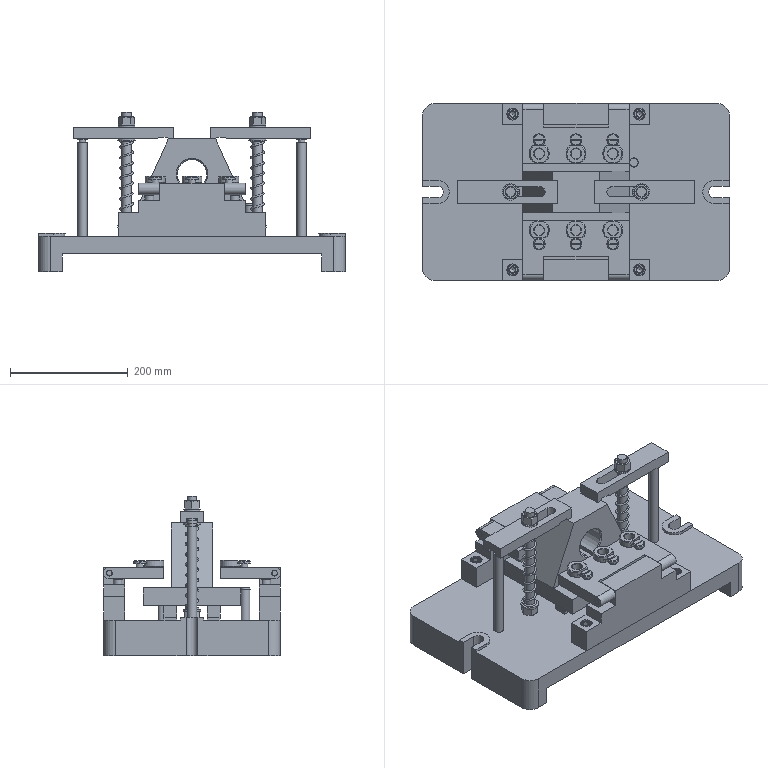Assembly | NX | mm | 56 component files | 56 solids | 875 faces | box 520 x 300 x 270 mm | volume 9321854 mm3 | plane 442 | cone 218 | cylinder 187 | torus 16 | spline 10 | sphere 2 | commonest cylinder face diameters 8 x22 16 x20 17 x20 26 x18 20 x16 10 x16 12 x8 11.701 x8
Bill of materials:
GB-T6170_F-2000,M16x2 | 4 |  | Hexagonal nut-like prism with a central circular through-bore, chamfered corners on both end faces and a chamfer at the bore entry.
unnamed part 1 | 4 |  | Solid stepped cylindrical pin: a large chamfered cylindrical head, a narrow undercut neck, and a smaller chamfered cylindrical shank.
unnamed part 2 | 6 |  | Slotted-head stepped fastener-like part: a chamfered round head with a straight screwdriver-style slot across it, a cylindrical shoulder, an undercut neck, and a smaller chamfered shank.
GB-T119.1-2000,8x40 | 2 |  | Parallel Pin, GB-T 119.1-2000,8x40
GB-T70.1-2000,M10x20 | 4 |  | Hexagon Socket Head Cap Screw, GB-T 70.1-2000,M10x20
unnamed part 3 | 6 |  | Flanged cylindrical bushing with a central through-bore. Part of one side of the flange is cut down to a lower step or flat.
GB-T848-2002,M16 | 2 |  | Flat annular ring (plain washer-like disc): a thin, uniform-thickness circular plate with a single concentric through-hole.
unnamed part 4 | 2 |  | Flat rectangular bar with a straight, round-ended slot cut through it toward one end, and a small trapezoidal groove across the underside near that end.
unnamed part 5 | 2 |  | Long rectangular block with symmetric stepped top levels: a raised central section, intermediate steps, and lower end pads. There are vertical holes in the end pads and the steps, and a small horizontal hole in an end face of the raised section.
unnamed part 6 | 2 |  | Rectangular bar with three vertical through-holes along its centerline: two larger holes near the ends and a smaller hole in the middle.
unnamed part 7 | 2 |  | Plain solid cylindrical rod with flat ends and no visible features.
unnamed part 8 | 2 |  | Helical coil spring made of round wire, with roughly ten open coils of constant diameter and pitch, apparently closed or flattened at the end turns.
GB-T70.1-2000,M12x40 | 4 |  | Hexagon Socket Head Cap Screw, GB-T 70.1-2000,M12x40
unnamed part 9 | 2 |  | Flat rectangular plate with a wide rectangular notch cut into one long edge, leaving two lugs. Each lug has a rounded end and a cross-hole running parallel to the plate. Three large and three small vertical holes are arranged in a row along the opposite edge.
unnamed part 10 | 2 |  | Slender cylindrical pin with a domed head at one end and a narrow circumferential groove just below the head. The rest of the shank is plain.
GB-T95-2002,M16 | 4 |  | Plain Washer, GB-T 95-2002,M16
unnamed part 11 | 1 |  | Rectangular base plate with rounded corners and two downward legs or rails along its short ends, giving a shallow channel-shaped profile. Each short edge has an open U-slot, and the top has two thin parallel raised strips. Many holes are spread over the plate: through-holes along the centerline and smaller holes near the strips and edges.
unnamed part 12 | 1 |  | Rectangular flat base plate with a single tapered (trapezoidal-profile) upright block centered on it. A circular through-bore with one rectangular keyway-style notch runs horizontally through the upright. Six through-holes in two rows of three go through the base plate, one row on each side of the upright.
GB-T119.1-2000,10x95 | 2 |  | Parallel Pin, GB-T 119.1-2000,10x95
GB-T119.1-2000,16x75 | 2 |  | Parallel Pin, GB-T 119.1-2000,16x75
Mates:
1. fix | fixture_body 1 component
2. center | bracket 1 face | bracket 1 face | fixture_body 1 face | fixture_body 1 face
3. touch align | datum_block 2 face | fixture_body 1 face
4. touch align | datum_block 2 face | fixture_body 1 face
5. touch align | datum_block 2 face | fixture_body 1 face
6. bond | datum_block 2 component | assembly component
7. bond | datum_block 2 component | assembly component
8. bond | datum_block 1 component | assembly component
9. linear | assembly datumaxis | assembly cartesiancoordinatesystem | assembly cartesiancoordinatesystem
10. touch align | datum_block 2 face | bracket 1 face
11. center | bracket 1 face | bracket 1 face | datum_block 2 face | datum_block 2 face
12. touch align | clamp_plate 2 face | bracket 1 face
13. center | clamp_plate 2 face | clamp_plate 2 face | bracket 1 face | bracket 1 face
14. touch align | stud_A 2 face | clamp_plate 2 face
15. distance | stud_A 2 face | fixture_body 1 face
16. distance | stud_B 2 face | fixture_body 1 face
17. touch align | stud_A 2 face | fixture_body 1 face
18. touch align | stud_B 2 face | fixture_body 1 face
19. bond | bracket 1 component | assembly component
20. bond | clamp_plate 2 component | assembly component
21. bond | stud_A 2 component | assembly component
22. bond | stud_B 2 component | assembly component
23. bond | clamp_plate 1 component | assembly component
24. bond | stud_A 1 component | assembly component
25. bond | stud_B 1 component | assembly component
26. circular | assembly datumaxis | assembly cartesiancoordinatesystem | assembly cartesiancoordinatesystem
27. circular | assembly datumaxis | assembly cartesiancoordinatesystem | assembly cartesiancoordinatesystem
28. circular | assembly datumaxis | assembly cartesiancoordinatesystem | assembly cartesiancoordinatesystem
29. concentric | GB-T6170_F-2000_M16x2 4 edge | fixture_body 1 arc
30. concentric | GB-T95-2002_M16 4 edge | GB-T6170_F-2000_M16x2 4 edge
31. touch align | GB-T95-2002_M16 3 face | stud_A 2 face
32. touch align | GB-T95-2002_M16 3 face | clamp_plate 2 face
33. concentric | GB-T848-2002_M16 2 edge | clamp_plate 2 edge
34. concentric | GB-T6170_F-2000_M16x2 3 edge | GB-T848-2002_M16 2 edge
35. concentric | spring 2 edge | GB-T95-2002_M16 4 edge
36. bond | GB-T6170_F-2000_M16x2 4 component | assembly component
37. bond | GB-T6170_F-2000_M16x2 2 component | assembly component
38. circular | assembly datumaxis | assembly cartesiancoordinatesystem | assembly cartesiancoordinatesystem
39. bond | GB-T95-2002_M16 4 component | assembly component
40. bond | GB-T95-2002_M16 2 component | assembly component
41. circular | assembly datumaxis | assembly cartesiancoordinatesystem | assembly cartesiancoordinatesystem
42. bond | GB-T6170_F-2000_M16x2 3 component | assembly component
43. bond | GB-T6170_F-2000_M16x2 1 component | assembly component
44. circular | assembly datumaxis | assembly cartesiancoordinatesystem | assembly cartesiancoordinatesystem
45. bond | GB-T848-2002_M16 2 component | assembly component
46. bond | GB-T848-2002_M16 1 component | assembly component
47. circular | assembly datumaxis | assembly cartesiancoordinatesystem | assembly cartesiancoordinatesystem
48. concentric | spring 1 edge | GB-T95-2002_M16 2 edge
49. concentric | GB-T119_1-2000_16x75 2 edge | fixture_body 1 edge
50. concentric | GB-T119_1-2000_16x75 1 edge | fixture_body 1 edge
51. touch align | support 2 face | fixture_body 1 face
52. touch align | support 2 face | fixture_body 1 face
53. center | support 2 face | support 2 face | bracket 1 face | bracket 1 face
54. bond | support 2 component | assembly component
55. bond | support 1 component | assembly component
56. circular | assembly datumaxis | assembly cartesiancoordinatesystem | assembly cartesiancoordinatesystem
57. touch align | drill_template 2 face | bracket 1 face
58. concentric | drill_bush 6 edge | drill_template 2 edge
59. touch align | drill_template 2 face | support 1 face
60. concentric | support_pin 4 edge | support 1 edge
61. concentric | support_pin 3 edge | support 1 edge
62. concentric | drill_bush_screw 6 edge | drill_template 2 arc
63. bond | drill_template 2 component | assembly component
64. bond | drill_bush 6 component | assembly component
65. bond | drill_bush_screw 6 component | assembly component
66. bond | drill_bush 5 component | assembly component
67. bond | drill_bush_screw 5 component | assembly component
68. linear | assembly datumaxis | assembly cartesiancoordinatesystem | assembly cartesiancoordinatesystem | assembly cartesiancoordinatesystem
69. linear | assembly datumaxis | assembly cartesiancoordinatesystem | assembly cartesiancoordinatesystem | assembly cartesiancoordinatesystem
70. bond | drill_bush 4 component | assembly component
71. bond | drill_bush_screw 4 component | assembly component
72. bond | drill_bush 4 component | assembly component
73. bond | drill_bush 3 component | assembly component
74. circular | assembly datumaxis | assembly cartesiancoordinatesystem | assembly cartesiancoordinatesystem
75. bond | drill_bush_screw 4 component | assembly component
76. bond | drill_bush_screw 3 component | assembly component
77. circular | assembly datumaxis | assembly cartesiancoordinatesystem | assembly cartesiancoordinatesystem
78. bond | drill_bush 5 component | assembly component
79. bond | drill_bush 2 component | assembly component
80. circular | assembly datumaxis | assembly cartesiancoordinatesystem | assembly cartesiancoordinatesystem
81. bond | drill_bush_screw 5 component | assembly component
82. bond | drill_bush_screw 2 component | assembly component
83. circular | assembly datumaxis | assembly cartesiancoordinatesystem | assembly cartesiancoordinatesystem
84. bond | drill_bush 6 component | assembly component
85. bond | drill_bush 1 component | assembly component
86. circular | assembly datumaxis | assembly cartesiancoordinatesystem | assembly cartesiancoordinatesystem
87. bond | drill_bush_screw 6 component | assembly component
88. bond | drill_bush_screw 1 component | assembly component
89. circular | assembly datumaxis | assembly cartesiancoordinatesystem | assembly cartesiancoordinatesystem
90. bond | drill_template 2 component | assembly component
91. bond | drill_template 1 component | assembly component
92. circular | assembly datumaxis | assembly cartesiancoordinatesystem | assembly cartesiancoordinatesystem
93. bond | support_pin 4 component | assembly component
94. bond | support_pin 2 component | assembly component
95. circular | assembly datumaxis | assembly cartesiancoordinatesystem | assembly cartesiancoordinatesystem
96. bond | support_pin 3 component | assembly component
97. bond | support_pin 1 component | assembly component
98. circular | assembly datumaxis | assembly cartesiancoordinatesystem | assembly cartesiancoordinatesystem
99. bond | hinge 2 component | assembly component
100. bond | hinge 1 component | assembly component
101. circular | assembly datumaxis | assembly cartesiancoordinatesystem | assembly cartesiancoordinatesystem
102. bond | GB-T70_1-2000_M12x40 3 component | assembly component
103. bond | GB-T70_1-2000_M12x40 2 component | assembly component
104. circular | assembly datumaxis | assembly cartesiancoordinatesystem | assembly cartesiancoordinatesystem
105. bond | GB-T70_1-2000_M12x40 4 component | assembly component
106. bond | GB-T70_1-2000_M12x40 1 component | assembly component
107. circular | assembly datumaxis | assembly cartesiancoordinatesystem | assembly cartesiancoordinatesystem
108. bond | GB-T95-2002_M16 3 component | assembly component
109. bond | GB-T95-2002_M16 1 component | assembly component
110. circular | assembly datumaxis | assembly cartesiancoordinatesystem | assembly cartesiancoordinatesystem